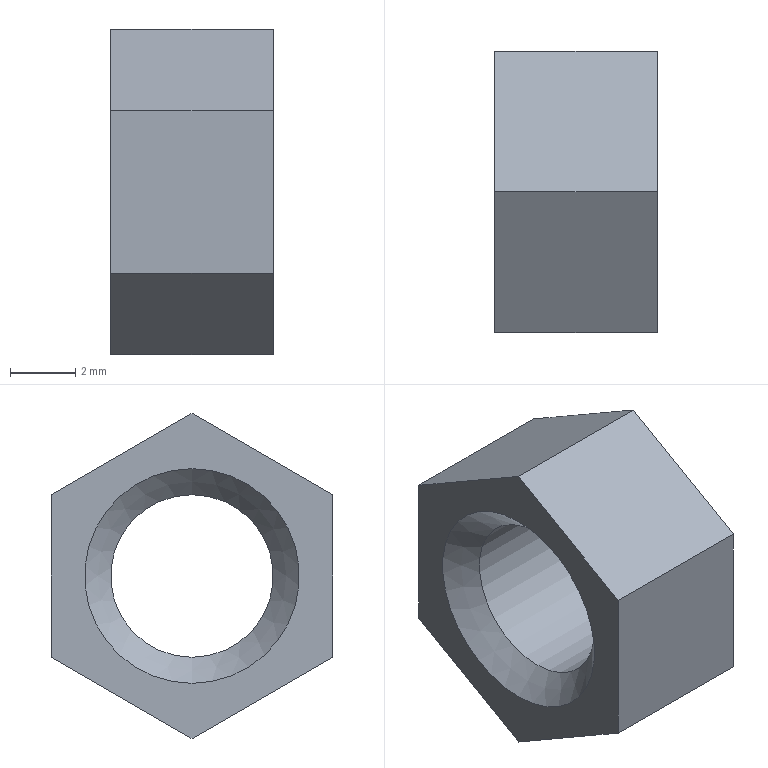Component | NX | ASSY_PRAC_PART_4 | 1 solid | 11 faces | box 5 x 8.66 x 10 mm | volume 215 mm3 | plane 8 | cone 2 | cylinder 1 | commonest cylinder face diameters 5 x1
STEP:
#1=CARTESIAN_POINT('',(0.,0.,0.));
#2=DIRECTION('',(0.,0.,1.));
#3=DIRECTION('',(1.,0.,0.));
#4=AXIS2_PLACEMENT_3D('',#1,#2,#3);
#5=CARTESIAN_POINT('',(18.5,0.3851,25.561));
#6=VERTEX_POINT('',#5);
#7=CARTESIAN_POINT('',(18.5,-3.945,23.061));
#8=VERTEX_POINT('',#7);
#9=CARTESIAN_POINT('',(18.5,0.3851,25.561));
#10=DIRECTION('',(0.,-0.866,-0.5));
#11=VECTOR('',#10,1.);
#12=LINE('',#9,#11);
#13=CARTESIAN_POINT('',(23.5,0.3851,25.561));
#14=DIRECTION('',(0.,0.5,-0.866));
#15=DIRECTION('',(0.,0.866,0.5));
#16=AXIS2_PLACEMENT_3D('',#13,#14,#15);
#17=PLANE('',#16);
#18=CARTESIAN_POINT('',(0.,-5.));
#19=DIRECTION('',(-1.,0.));
#20=VECTOR('',#19,1.);
#21=LINE('',#18,#20);
#22=(GEOMETRIC_REPRESENTATION_CONTEXT(2)PARAMETRIC_REPRESENTATION_CONTEXT()REPRESENTATION_CONTEXT('',''));
#23=DEFINITIONAL_REPRESENTATION('',(#21),#22);
#24=PCURVE('',#17,#23);
#25=CARTESIAN_POINT('',(18.5,0.3851,20.561));
#26=DIRECTION('',(1.,0.,0.));
#27=DIRECTION('',(0.,0.,-1.));
#28=AXIS2_PLACEMENT_3D('',#25,#26,#27);
#29=PLANE('',#28);
#30=CARTESIAN_POINT('',(-5.,0.));
#31=DIRECTION('',(0.5,-0.866));
#32=VECTOR('',#31,1.);
#33=LINE('',#30,#32);
#34=(GEOMETRIC_REPRESENTATION_CONTEXT(2)PARAMETRIC_REPRESENTATION_CONTEXT()REPRESENTATION_CONTEXT('',''));
#35=DEFINITIONAL_REPRESENTATION('',(#33),#34);
#36=PCURVE('',#29,#35);
#37=SURFACE_CURVE('',#12,(#24,#36),.PCURVE_S1.);
#38=EDGE_CURVE('',#6,#8,#37,.T.);
#39=ORIENTED_EDGE('',*,*,#38,.T.);
#40=CARTESIAN_POINT('',(23.5,-3.945,23.061));
#41=VERTEX_POINT('',#40);
#42=CARTESIAN_POINT('',(23.5,-3.945,23.061));
#43=DIRECTION('',(-1.,0.,0.));
#44=VECTOR('',#43,1.);
#45=LINE('',#42,#44);
#46=CARTESIAN_POINT('',(-5.,0.));
#47=DIRECTION('',(0.,-1.));
#48=VECTOR('',#47,1.);
#49=LINE('',#46,#48);
#50=(GEOMETRIC_REPRESENTATION_CONTEXT(2)PARAMETRIC_REPRESENTATION_CONTEXT()REPRESENTATION_CONTEXT('',''));
#51=DEFINITIONAL_REPRESENTATION('',(#49),#50);
#52=PCURVE('',#17,#51);
#53=CARTESIAN_POINT('',(23.5,-3.945,23.061));
#54=DIRECTION('',(0.,1.,-0.));
#55=DIRECTION('',(0.,0.,1.));
#56=AXIS2_PLACEMENT_3D('',#53,#54,#55);
#57=PLANE('',#56);
#58=CARTESIAN_POINT('',(0.,0.));
#59=DIRECTION('',(0.,-1.));
#60=VECTOR('',#59,1.);
#61=LINE('',#58,#60);
#62=(GEOMETRIC_REPRESENTATION_CONTEXT(2)PARAMETRIC_REPRESENTATION_CONTEXT()REPRESENTATION_CONTEXT('',''));
#63=DEFINITIONAL_REPRESENTATION('',(#61),#62);
#64=PCURVE('',#57,#63);
#65=SURFACE_CURVE('',#45,(#52,#64),.PCURVE_S1.);
#66=EDGE_CURVE('',#41,#8,#65,.T.);
#67=ORIENTED_EDGE('',*,*,#66,.F.);
#68=CARTESIAN_POINT('',(23.5,0.3851,25.561));
#69=VERTEX_POINT('',#68);
#70=CARTESIAN_POINT('',(23.5,0.3851,25.561));
#71=DIRECTION('',(0.,-0.866,-0.5));
#72=VECTOR('',#71,1.);
#73=LINE('',#70,#72);
#74=CARTESIAN_POINT('',(0.,0.));
#75=DIRECTION('',(-1.,0.));
#76=VECTOR('',#75,1.);
#77=LINE('',#74,#76);
#78=(GEOMETRIC_REPRESENTATION_CONTEXT(2)PARAMETRIC_REPRESENTATION_CONTEXT()REPRESENTATION_CONTEXT('',''));
#79=DEFINITIONAL_REPRESENTATION('',(#77),#78);
#80=PCURVE('',#17,#79);
#81=CARTESIAN_POINT('',(23.5,0.3851,20.561));
#82=DIRECTION('',(1.,0.,0.));
#83=DIRECTION('',(0.,0.,-1.));
#84=AXIS2_PLACEMENT_3D('',#81,#82,#83);
#85=PLANE('',#84);
#86=CARTESIAN_POINT('',(-5.,0.));
#87=DIRECTION('',(0.5,-0.866));
#88=VECTOR('',#87,1.);
#89=LINE('',#86,#88);
#90=(GEOMETRIC_REPRESENTATION_CONTEXT(2)PARAMETRIC_REPRESENTATION_CONTEXT()REPRESENTATION_CONTEXT('',''));
#91=DEFINITIONAL_REPRESENTATION('',(#89),#90);
#92=PCURVE('',#85,#91);
#93=SURFACE_CURVE('',#73,(#80,#92),.PCURVE_S1.);
#94=EDGE_CURVE('',#69,#41,#93,.T.);
#95=ORIENTED_EDGE('',*,*,#94,.F.);
#96=CARTESIAN_POINT('',(23.5,0.3851,25.561));
#97=DIRECTION('',(-1.,0.,0.));
#98=VECTOR('',#97,1.);
#99=LINE('',#96,#98);
#100=CARTESIAN_POINT('',(0.,0.));
#101=DIRECTION('',(0.,-1.));
#102=VECTOR('',#101,1.);
#103=LINE('',#100,#102);
#104=(GEOMETRIC_REPRESENTATION_CONTEXT(2)PARAMETRIC_REPRESENTATION_CONTEXT()REPRESENTATION_CONTEXT('',''));
#105=DEFINITIONAL_REPRESENTATION('',(#103),#104);
#106=PCURVE('',#17,#105);
#107=CARTESIAN_POINT('',(23.5,4.715,23.061));
#108=DIRECTION('',(0.,-0.5,-0.866));
#109=DIRECTION('',(0.,0.866,-0.5));
#110=AXIS2_PLACEMENT_3D('',#107,#108,#109);
#111=PLANE('',#110);
#112=CARTESIAN_POINT('',(-5.,0.));
#113=DIRECTION('',(0.,-1.));
#114=VECTOR('',#113,1.);
#115=LINE('',#112,#114);
#116=(GEOMETRIC_REPRESENTATION_CONTEXT(2)PARAMETRIC_REPRESENTATION_CONTEXT()REPRESENTATION_CONTEXT('',''));
#117=DEFINITIONAL_REPRESENTATION('',(#115),#116);
#118=PCURVE('',#111,#117);
#119=SURFACE_CURVE('',#99,(#106,#118),.PCURVE_S1.);
#120=EDGE_CURVE('',#69,#6,#119,.T.);
#121=ORIENTED_EDGE('',*,*,#120,.T.);
#122=EDGE_LOOP('',(#39,#67,#95,#121));
#123=FACE_BOUND('',#122,.T.);
#124=ADVANCED_FACE('',(#123),#17,.F.);
#125=CARTESIAN_POINT('',(18.5,-3.945,18.061));
#126=VERTEX_POINT('',#125);
#127=CARTESIAN_POINT('',(18.5,-3.945,23.061));
#128=DIRECTION('',(0.,-0.,-1.));
#129=VECTOR('',#128,1.);
#130=LINE('',#127,#129);
#131=CARTESIAN_POINT('',(0.,-5.));
#132=DIRECTION('',(-1.,0.));
#133=VECTOR('',#132,1.);
#134=LINE('',#131,#133);
#135=(GEOMETRIC_REPRESENTATION_CONTEXT(2)PARAMETRIC_REPRESENTATION_CONTEXT()REPRESENTATION_CONTEXT('',''));
#136=DEFINITIONAL_REPRESENTATION('',(#134),#135);
#137=PCURVE('',#57,#136);
#138=CARTESIAN_POINT('',(-2.5,-4.33));
#139=DIRECTION('',(1.,-0.));
#140=VECTOR('',#139,1.);
#141=LINE('',#138,#140);
#142=(GEOMETRIC_REPRESENTATION_CONTEXT(2)PARAMETRIC_REPRESENTATION_CONTEXT()REPRESENTATION_CONTEXT('',''));
#143=DEFINITIONAL_REPRESENTATION('',(#141),#142);
#144=PCURVE('',#29,#143);
#145=SURFACE_CURVE('',#130,(#137,#144),.PCURVE_S1.);
#146=EDGE_CURVE('',#8,#126,#145,.T.);
#147=ORIENTED_EDGE('',*,*,#146,.T.);
#148=CARTESIAN_POINT('',(23.5,-3.945,18.061));
#149=VERTEX_POINT('',#148);
#150=CARTESIAN_POINT('',(23.5,-3.945,18.061));
#151=DIRECTION('',(-1.,0.,0.));
#152=VECTOR('',#151,1.);
#153=LINE('',#150,#152);
#154=CARTESIAN_POINT('',(-5.,0.));
#155=DIRECTION('',(0.,-1.));
#156=VECTOR('',#155,1.);
#157=LINE('',#154,#156);
#158=(GEOMETRIC_REPRESENTATION_CONTEXT(2)PARAMETRIC_REPRESENTATION_CONTEXT()REPRESENTATION_CONTEXT('',''));
#159=DEFINITIONAL_REPRESENTATION('',(#157),#158);
#160=PCURVE('',#57,#159);
#161=CARTESIAN_POINT('',(23.5,-3.945,18.061));
#162=DIRECTION('',(0.,0.5,0.866));
#163=DIRECTION('',(0.,-0.866,0.5));
#164=AXIS2_PLACEMENT_3D('',#161,#162,#163);
#165=PLANE('',#164);
#166=CARTESIAN_POINT('',(0.,0.));
#167=DIRECTION('',(0.,-1.));
#168=VECTOR('',#167,1.);
#169=LINE('',#166,#168);
#170=(GEOMETRIC_REPRESENTATION_CONTEXT(2)PARAMETRIC_REPRESENTATION_CONTEXT()REPRESENTATION_CONTEXT('',''));
#171=DEFINITIONAL_REPRESENTATION('',(#169),#170);
#172=PCURVE('',#165,#171);
#173=SURFACE_CURVE('',#153,(#160,#172),.PCURVE_S1.);
#174=EDGE_CURVE('',#149,#126,#173,.T.);
#175=ORIENTED_EDGE('',*,*,#174,.F.);
#176=CARTESIAN_POINT('',(23.5,-3.945,23.061));
#177=DIRECTION('',(0.,-0.,-1.));
#178=VECTOR('',#177,1.);
#179=LINE('',#176,#178);
#180=CARTESIAN_POINT('',(0.,0.));
#181=DIRECTION('',(-1.,0.));
#182=VECTOR('',#181,1.);
#183=LINE('',#180,#182);
#184=(GEOMETRIC_REPRESENTATION_CONTEXT(2)PARAMETRIC_REPRESENTATION_CONTEXT()REPRESENTATION_CONTEXT('',''));
#185=DEFINITIONAL_REPRESENTATION('',(#183),#184);
#186=PCURVE('',#57,#185);
#187=CARTESIAN_POINT('',(-2.5,-4.33));
#188=DIRECTION('',(1.,-0.));
#189=VECTOR('',#188,1.);
#190=LINE('',#187,#189);
#191=(GEOMETRIC_REPRESENTATION_CONTEXT(2)PARAMETRIC_REPRESENTATION_CONTEXT()REPRESENTATION_CONTEXT('',''));
#192=DEFINITIONAL_REPRESENTATION('',(#190),#191);
#193=PCURVE('',#85,#192);
#194=SURFACE_CURVE('',#179,(#186,#193),.PCURVE_S1.);
#195=EDGE_CURVE('',#41,#149,#194,.T.);
#196=ORIENTED_EDGE('',*,*,#195,.F.);
#197=ORIENTED_EDGE('',*,*,#66,.T.);
#198=EDGE_LOOP('',(#147,#175,#196,#197));
#199=FACE_BOUND('',#198,.T.);
#200=ADVANCED_FACE('',(#199),#57,.F.);
#201=CARTESIAN_POINT('',(18.5,0.3851,15.561));
#202=VERTEX_POINT('',#201);
#203=CARTESIAN_POINT('',(18.5,-3.945,18.061));
#204=DIRECTION('',(0.,0.866,-0.5));
#205=VECTOR('',#204,1.);
#206=LINE('',#203,#205);
#207=CARTESIAN_POINT('',(0.,-5.));
#208=DIRECTION('',(-1.,0.));
#209=VECTOR('',#208,1.);
#210=LINE('',#207,#209);
#211=(GEOMETRIC_REPRESENTATION_CONTEXT(2)PARAMETRIC_REPRESENTATION_CONTEXT()REPRESENTATION_CONTEXT('',''));
#212=DEFINITIONAL_REPRESENTATION('',(#210),#211);
#213=PCURVE('',#165,#212);
#214=CARTESIAN_POINT('',(2.5,-4.33));
#215=DIRECTION('',(0.5,0.866));
#216=VECTOR('',#215,1.);
#217=LINE('',#214,#216);
#218=(GEOMETRIC_REPRESENTATION_CONTEXT(2)PARAMETRIC_REPRESENTATION_CONTEXT()REPRESENTATION_CONTEXT('',''));
#219=DEFINITIONAL_REPRESENTATION('',(#217),#218);
#220=PCURVE('',#29,#219);
#221=SURFACE_CURVE('',#206,(#213,#220),.PCURVE_S1.);
#222=EDGE_CURVE('',#126,#202,#221,.T.);
#223=ORIENTED_EDGE('',*,*,#222,.T.);
#224=CARTESIAN_POINT('',(23.5,0.3851,15.561));
#225=VERTEX_POINT('',#224);
#226=CARTESIAN_POINT('',(23.5,0.3851,15.561));
#227=DIRECTION('',(-1.,0.,0.));
#228=VECTOR('',#227,1.);
#229=LINE('',#226,#228);
#230=CARTESIAN_POINT('',(-5.,0.));
#231=DIRECTION('',(0.,-1.));
#232=VECTOR('',#231,1.);
#233=LINE('',#230,#232);
#234=(GEOMETRIC_REPRESENTATION_CONTEXT(2)PARAMETRIC_REPRESENTATION_CONTEXT()REPRESENTATION_CONTEXT('',''));
#235=DEFINITIONAL_REPRESENTATION('',(#233),#234);
#236=PCURVE('',#165,#235);
#237=CARTESIAN_POINT('',(23.5,0.3851,15.561));
#238=DIRECTION('',(0.,-0.5,0.866));
#239=DIRECTION('',(0.,-0.866,-0.5));
#240=AXIS2_PLACEMENT_3D('',#237,#238,#239);
#241=PLANE('',#240);
#242=CARTESIAN_POINT('',(0.,0.));
#243=DIRECTION('',(0.,-1.));
#244=VECTOR('',#243,1.);
#245=LINE('',#242,#244);
#246=(GEOMETRIC_REPRESENTATION_CONTEXT(2)PARAMETRIC_REPRESENTATION_CONTEXT()REPRESENTATION_CONTEXT('',''));
#247=DEFINITIONAL_REPRESENTATION('',(#245),#246);
#248=PCURVE('',#241,#247);
#249=SURFACE_CURVE('',#229,(#236,#248),.PCURVE_S1.);
#250=EDGE_CURVE('',#225,#202,#249,.T.);
#251=ORIENTED_EDGE('',*,*,#250,.F.);
#252=CARTESIAN_POINT('',(23.5,-3.945,18.061));
#253=DIRECTION('',(0.,0.866,-0.5));
#254=VECTOR('',#253,1.);
#255=LINE('',#252,#254);
#256=CARTESIAN_POINT('',(0.,0.));
#257=DIRECTION('',(-1.,0.));
#258=VECTOR('',#257,1.);
#259=LINE('',#256,#258);
#260=(GEOMETRIC_REPRESENTATION_CONTEXT(2)PARAMETRIC_REPRESENTATION_CONTEXT()REPRESENTATION_CONTEXT('',''));
#261=DEFINITIONAL_REPRESENTATION('',(#259),#260);
#262=PCURVE('',#165,#261);
#263=CARTESIAN_POINT('',(2.5,-4.33));
#264=DIRECTION('',(0.5,0.866));
#265=VECTOR('',#264,1.);
#266=LINE('',#263,#265);
#267=(GEOMETRIC_REPRESENTATION_CONTEXT(2)PARAMETRIC_REPRESENTATION_CONTEXT()REPRESENTATION_CONTEXT('',''));
#268=DEFINITIONAL_REPRESENTATION('',(#266),#267);
#269=PCURVE('',#85,#268);
#270=SURFACE_CURVE('',#255,(#262,#269),.PCURVE_S1.);
#271=EDGE_CURVE('',#149,#225,#270,.T.);
#272=ORIENTED_EDGE('',*,*,#271,.F.);
#273=ORIENTED_EDGE('',*,*,#174,.T.);
#274=EDGE_LOOP('',(#223,#251,#272,#273));
#275=FACE_BOUND('',#274,.T.);
#276=ADVANCED_FACE('',(#275),#165,.F.);
#277=CARTESIAN_POINT('',(18.5,4.715,18.061));
#278=VERTEX_POINT('',#277);
#279=CARTESIAN_POINT('',(18.5,0.3851,15.561));
#280=DIRECTION('',(0.,0.866,0.5));
#281=VECTOR('',#280,1.);
#282=LINE('',#279,#281);
#283=CARTESIAN_POINT('',(0.,-5.));
#284=DIRECTION('',(-1.,0.));
#285=VECTOR('',#284,1.);
#286=LINE('',#283,#285);
#287=(GEOMETRIC_REPRESENTATION_CONTEXT(2)PARAMETRIC_REPRESENTATION_CONTEXT()REPRESENTATION_CONTEXT('',''));
#288=DEFINITIONAL_REPRESENTATION('',(#286),#287);
#289=PCURVE('',#241,#288);
#290=CARTESIAN_POINT('',(5.,-0.));
#291=DIRECTION('',(-0.5,0.866));
#292=VECTOR('',#291,1.);
#293=LINE('',#290,#292);
#294=(GEOMETRIC_REPRESENTATION_CONTEXT(2)PARAMETRIC_REPRESENTATION_CONTEXT()REPRESENTATION_CONTEXT('',''));
#295=DEFINITIONAL_REPRESENTATION('',(#293),#294);
#296=PCURVE('',#29,#295);
#297=SURFACE_CURVE('',#282,(#289,#296),.PCURVE_S1.);
#298=EDGE_CURVE('',#202,#278,#297,.T.);
#299=ORIENTED_EDGE('',*,*,#298,.T.);
#300=CARTESIAN_POINT('',(23.5,4.715,18.061));
#301=VERTEX_POINT('',#300);
#302=CARTESIAN_POINT('',(23.5,4.715,18.061));
#303=DIRECTION('',(-1.,0.,0.));
#304=VECTOR('',#303,1.);
#305=LINE('',#302,#304);
#306=CARTESIAN_POINT('',(-5.,0.));
#307=DIRECTION('',(0.,-1.));
#308=VECTOR('',#307,1.);
#309=LINE('',#306,#308);
#310=(GEOMETRIC_REPRESENTATION_CONTEXT(2)PARAMETRIC_REPRESENTATION_CONTEXT()REPRESENTATION_CONTEXT('',''));
#311=DEFINITIONAL_REPRESENTATION('',(#309),#310);
#312=PCURVE('',#241,#311);
#313=CARTESIAN_POINT('',(23.5,4.715,18.061));
#314=DIRECTION('',(0.,-1.,0.));
#315=DIRECTION('',(0.,-0.,-1.));
#316=AXIS2_PLACEMENT_3D('',#313,#314,#315);
#317=PLANE('',#316);
#318=CARTESIAN_POINT('',(0.,0.));
#319=DIRECTION('',(0.,-1.));
#320=VECTOR('',#319,1.);
#321=LINE('',#318,#320);
#322=(GEOMETRIC_REPRESENTATION_CONTEXT(2)PARAMETRIC_REPRESENTATION_CONTEXT()REPRESENTATION_CONTEXT('',''));
#323=DEFINITIONAL_REPRESENTATION('',(#321),#322);
#324=PCURVE('',#317,#323);
#325=SURFACE_CURVE('',#305,(#312,#324),.PCURVE_S1.);
#326=EDGE_CURVE('',#301,#278,#325,.T.);
#327=ORIENTED_EDGE('',*,*,#326,.F.);
#328=CARTESIAN_POINT('',(23.5,0.3851,15.561));
#329=DIRECTION('',(0.,0.866,0.5));
#330=VECTOR('',#329,1.);
#331=LINE('',#328,#330);
#332=CARTESIAN_POINT('',(0.,0.));
#333=DIRECTION('',(-1.,0.));
#334=VECTOR('',#333,1.);
#335=LINE('',#332,#334);
#336=(GEOMETRIC_REPRESENTATION_CONTEXT(2)PARAMETRIC_REPRESENTATION_CONTEXT()REPRESENTATION_CONTEXT('',''));
#337=DEFINITIONAL_REPRESENTATION('',(#335),#336);
#338=PCURVE('',#241,#337);
#339=CARTESIAN_POINT('',(5.,-0.));
#340=DIRECTION('',(-0.5,0.866));
#341=VECTOR('',#340,1.);
#342=LINE('',#339,#341);
#343=(GEOMETRIC_REPRESENTATION_CONTEXT(2)PARAMETRIC_REPRESENTATION_CONTEXT()REPRESENTATION_CONTEXT('',''));
#344=DEFINITIONAL_REPRESENTATION('',(#342),#343);
#345=PCURVE('',#85,#344);
#346=SURFACE_CURVE('',#331,(#338,#345),.PCURVE_S1.);
#347=EDGE_CURVE('',#225,#301,#346,.T.);
#348=ORIENTED_EDGE('',*,*,#347,.F.);
#349=ORIENTED_EDGE('',*,*,#250,.T.);
#350=EDGE_LOOP('',(#299,#327,#348,#349));
#351=FACE_BOUND('',#350,.T.);
#352=ADVANCED_FACE('',(#351),#241,.F.);
#353=CARTESIAN_POINT('',(18.5,4.715,23.061));
#354=VERTEX_POINT('',#353);
#355=CARTESIAN_POINT('',(18.5,4.715,18.061));
#356=DIRECTION('',(0.,0.,1.));
#357=VECTOR('',#356,1.);
#358=LINE('',#355,#357);
#359=CARTESIAN_POINT('',(0.,-5.));
#360=DIRECTION('',(-1.,0.));
#361=VECTOR('',#360,1.);
#362=LINE('',#359,#361);
#363=(GEOMETRIC_REPRESENTATION_CONTEXT(2)PARAMETRIC_REPRESENTATION_CONTEXT()REPRESENTATION_CONTEXT('',''));
#364=DEFINITIONAL_REPRESENTATION('',(#362),#363);
#365=PCURVE('',#317,#364);
#366=CARTESIAN_POINT('',(2.5,4.33));
#367=DIRECTION('',(-1.,0.));
#368=VECTOR('',#367,1.);
#369=LINE('',#366,#368);
#370=(GEOMETRIC_REPRESENTATION_CONTEXT(2)PARAMETRIC_REPRESENTATION_CONTEXT()REPRESENTATION_CONTEXT('',''));
#371=DEFINITIONAL_REPRESENTATION('',(#369),#370);
#372=PCURVE('',#29,#371);
#373=SURFACE_CURVE('',#358,(#365,#372),.PCURVE_S1.);
#374=EDGE_CURVE('',#278,#354,#373,.T.);
#375=ORIENTED_EDGE('',*,*,#374,.T.);
#376=CARTESIAN_POINT('',(23.5,4.715,23.061));
#377=VERTEX_POINT('',#376);
#378=CARTESIAN_POINT('',(23.5,4.715,23.061));
#379=DIRECTION('',(-1.,0.,0.));
#380=VECTOR('',#379,1.);
#381=LINE('',#378,#380);
#382=CARTESIAN_POINT('',(-5.,0.));
#383=DIRECTION('',(0.,-1.));
#384=VECTOR('',#383,1.);
#385=LINE('',#382,#384);
#386=(GEOMETRIC_REPRESENTATION_CONTEXT(2)PARAMETRIC_REPRESENTATION_CONTEXT()REPRESENTATION_CONTEXT('',''));
#387=DEFINITIONAL_REPRESENTATION('',(#385),#386);
#388=PCURVE('',#317,#387);
#389=CARTESIAN_POINT('',(0.,0.));
#390=DIRECTION('',(0.,-1.));
#391=VECTOR('',#390,1.);
#392=LINE('',#389,#391);
#393=(GEOMETRIC_REPRESENTATION_CONTEXT(2)PARAMETRIC_REPRESENTATION_CONTEXT()REPRESENTATION_CONTEXT('',''));
#394=DEFINITIONAL_REPRESENTATION('',(#392),#393);
#395=PCURVE('',#111,#394);
#396=SURFACE_CURVE('',#381,(#388,#395),.PCURVE_S1.);
#397=EDGE_CURVE('',#377,#354,#396,.T.);
#398=ORIENTED_EDGE('',*,*,#397,.F.);
#399=CARTESIAN_POINT('',(23.5,4.715,18.061));
#400=DIRECTION('',(0.,0.,1.));
#401=VECTOR('',#400,1.);
#402=LINE('',#399,#401);
#403=CARTESIAN_POINT('',(0.,0.));
#404=DIRECTION('',(-1.,0.));
#405=VECTOR('',#404,1.);
#406=LINE('',#403,#405);
#407=(GEOMETRIC_REPRESENTATION_CONTEXT(2)PARAMETRIC_REPRESENTATION_CONTEXT()REPRESENTATION_CONTEXT('',''));
#408=DEFINITIONAL_REPRESENTATION('',(#406),#407);
#409=PCURVE('',#317,#408);
#410=CARTESIAN_POINT('',(2.5,4.33));
#411=DIRECTION('',(-1.,0.));
#412=VECTOR('',#411,1.);
#413=LINE('',#410,#412);
#414=(GEOMETRIC_REPRESENTATION_CONTEXT(2)PARAMETRIC_REPRESENTATION_CONTEXT()REPRESENTATION_CONTEXT('',''));
#415=DEFINITIONAL_REPRESENTATION('',(#413),#414);
#416=PCURVE('',#85,#415);
#417=SURFACE_CURVE('',#402,(#409,#416),.PCURVE_S1.);
#418=EDGE_CURVE('',#301,#377,#417,.T.);
#419=ORIENTED_EDGE('',*,*,#418,.F.);
#420=ORIENTED_EDGE('',*,*,#326,.T.);
#421=EDGE_LOOP('',(#375,#398,#419,#420));
#422=FACE_BOUND('',#421,.T.);
#423=ADVANCED_FACE('',(#422),#317,.F.);
#424=CARTESIAN_POINT('',(18.5,4.715,23.061));
#425=DIRECTION('',(0.,-0.866,0.5));
#426=VECTOR('',#425,1.);
#427=LINE('',#424,#426);
#428=CARTESIAN_POINT('',(0.,-5.));
#429=DIRECTION('',(-1.,0.));
#430=VECTOR('',#429,1.);
#431=LINE('',#428,#430);
#432=(GEOMETRIC_REPRESENTATION_CONTEXT(2)PARAMETRIC_REPRESENTATION_CONTEXT()REPRESENTATION_CONTEXT('',''));
#433=DEFINITIONAL_REPRESENTATION('',(#431),#432);
#434=PCURVE('',#111,#433);
#435=CARTESIAN_POINT('',(-2.5,4.33));
#436=DIRECTION('',(-0.5,-0.866));
#437=VECTOR('',#436,1.);
#438=LINE('',#435,#437);
#439=(GEOMETRIC_REPRESENTATION_CONTEXT(2)PARAMETRIC_REPRESENTATION_CONTEXT()REPRESENTATION_CONTEXT('',''));
#440=DEFINITIONAL_REPRESENTATION('',(#438),#439);
#441=PCURVE('',#29,#440);
#442=SURFACE_CURVE('',#427,(#434,#441),.PCURVE_S1.);
#443=EDGE_CURVE('',#354,#6,#442,.T.);
#444=ORIENTED_EDGE('',*,*,#443,.T.);
#445=ORIENTED_EDGE('',*,*,#120,.F.);
#446=CARTESIAN_POINT('',(23.5,4.715,23.061));
#447=DIRECTION('',(0.,-0.866,0.5));
#448=VECTOR('',#447,1.);
#449=LINE('',#446,#448);
#450=CARTESIAN_POINT('',(0.,0.));
#451=DIRECTION('',(-1.,0.));
#452=VECTOR('',#451,1.);
#453=LINE('',#450,#452);
#454=(GEOMETRIC_REPRESENTATION_CONTEXT(2)PARAMETRIC_REPRESENTATION_CONTEXT()REPRESENTATION_CONTEXT('',''));
#455=DEFINITIONAL_REPRESENTATION('',(#453),#454);
#456=PCURVE('',#111,#455);
#457=CARTESIAN_POINT('',(-2.5,4.33));
#458=DIRECTION('',(-0.5,-0.866));
#459=VECTOR('',#458,1.);
#460=LINE('',#457,#459);
#461=(GEOMETRIC_REPRESENTATION_CONTEXT(2)PARAMETRIC_REPRESENTATION_CONTEXT()REPRESENTATION_CONTEXT('',''));
#462=DEFINITIONAL_REPRESENTATION('',(#460),#461);
#463=PCURVE('',#85,#462);
#464=SURFACE_CURVE('',#449,(#456,#463),.PCURVE_S1.);
#465=EDGE_CURVE('',#377,#69,#464,.T.);
#466=ORIENTED_EDGE('',*,*,#465,.F.);
#467=ORIENTED_EDGE('',*,*,#397,.T.);
#468=EDGE_LOOP('',(#444,#445,#466,#467));
#469=FACE_BOUND('',#468,.T.);
#470=ADVANCED_FACE('',(#469),#111,.F.);
#471=CARTESIAN_POINT('',(23.5,0.3851,17.261));
#472=VERTEX_POINT('',#471);
#473=CARTESIAN_POINT('',(23.5,0.3851,20.561));
#474=DIRECTION('',(-1.,0.,0.));
#475=DIRECTION('',(0.,0.,-1.));
#476=AXIS2_PLACEMENT_3D('',#473,#474,#475);
#477=CIRCLE('',#476,3.3);
#478=CARTESIAN_POINT('',(3.3,0.));
#479=CARTESIAN_POINT('',(3.3,-5.716));
#480=CARTESIAN_POINT('',(-1.65,-2.858));
#481=CARTESIAN_POINT('',(-6.6,-0.));
#482=CARTESIAN_POINT('',(-1.65,2.858));
#483=CARTESIAN_POINT('',(3.3,5.716));
#484=CARTESIAN_POINT('',(3.3,0.));
#485=(BOUNDED_CURVE()B_SPLINE_CURVE(2,(#478,#479,#480,#481,#482,#483,#484),.UNSPECIFIED.,.T.,.F.)B_SPLINE_CURVE_WITH_KNOTS((1,2,2,2,2,1),(-2.094,0.,2.094,4.189,6.283,8.378),.UNSPECIFIED.)CURVE()GEOMETRIC_REPRESENTATION_ITEM()RATIONAL_B_SPLINE_CURVE((1.,0.5,1.,0.5,1.,0.5,1.))REPRESENTATION_ITEM(''));
#486=(GEOMETRIC_REPRESENTATION_CONTEXT(2)PARAMETRIC_REPRESENTATION_CONTEXT()REPRESENTATION_CONTEXT('',''));
#487=DEFINITIONAL_REPRESENTATION('',(#485),#486);
#488=PCURVE('',#85,#487);
#489=CARTESIAN_POINT('',(22.7,0.3851,20.561));
#490=DIRECTION('',(1.,0.,0.));
#491=DIRECTION('',(0.,0.,-1.));
#492=AXIS2_PLACEMENT_3D('',#489,#490,#491);
#493=CONICAL_SURFACE('',#492,2.5,0.7854);
#494=CARTESIAN_POINT('',(6.283,0.8));
#495=DIRECTION('',(-1.,0.));
#496=VECTOR('',#495,1.);
#497=LINE('',#494,#496);
#498=(GEOMETRIC_REPRESENTATION_CONTEXT(2)PARAMETRIC_REPRESENTATION_CONTEXT()REPRESENTATION_CONTEXT('',''));
#499=DEFINITIONAL_REPRESENTATION('',(#497),#498);
#500=PCURVE('',#493,#499);
#501=SURFACE_CURVE('',#477,(#488,#500),.PCURVE_S1.);
#502=EDGE_CURVE('',#472,#472,#501,.T.);
#503=ORIENTED_EDGE('',*,*,#502,.T.);
#504=EDGE_LOOP('',(#503));
#505=FACE_BOUND('',#504,.T.);
#506=ORIENTED_EDGE('',*,*,#94,.T.);
#507=ORIENTED_EDGE('',*,*,#195,.T.);
#508=ORIENTED_EDGE('',*,*,#271,.T.);
#509=ORIENTED_EDGE('',*,*,#347,.T.);
#510=ORIENTED_EDGE('',*,*,#418,.T.);
#511=ORIENTED_EDGE('',*,*,#465,.T.);
#512=EDGE_LOOP('',(#506,#507,#508,#509,#510,#511));
#513=FACE_BOUND('',#512,.T.);
#514=ADVANCED_FACE('',(#505,#513),#85,.T.);
#515=CARTESIAN_POINT('',(18.5,0.3851,17.261));
#516=VERTEX_POINT('',#515);
#517=CARTESIAN_POINT('',(18.5,0.3851,20.561));
#518=DIRECTION('',(1.,0.,0.));
#519=DIRECTION('',(0.,0.,-1.));
#520=AXIS2_PLACEMENT_3D('',#517,#518,#519);
#521=CIRCLE('',#520,3.3);
#522=CARTESIAN_POINT('',(0.,0.));
#523=DIRECTION('',(1.,0.));
#524=AXIS2_PLACEMENT_2D('',#522,#523);
#525=CIRCLE('',#524,3.3);
#526=(GEOMETRIC_REPRESENTATION_CONTEXT(2)PARAMETRIC_REPRESENTATION_CONTEXT()REPRESENTATION_CONTEXT('',''));
#527=DEFINITIONAL_REPRESENTATION('',(#525),#526);
#528=PCURVE('',#29,#527);
#529=CARTESIAN_POINT('',(18.5,0.3851,20.561));
#530=DIRECTION('',(-1.,0.,0.));
#531=DIRECTION('',(0.,0.,1.));
#532=AXIS2_PLACEMENT_3D('',#529,#530,#531);
#533=CONICAL_SURFACE('',#532,3.3,0.7854);
#534=CARTESIAN_POINT('',(9.425,0.));
#535=DIRECTION('',(-1.,0.));
#536=VECTOR('',#535,1.);
#537=LINE('',#534,#536);
#538=(GEOMETRIC_REPRESENTATION_CONTEXT(2)PARAMETRIC_REPRESENTATION_CONTEXT()REPRESENTATION_CONTEXT('',''));
#539=DEFINITIONAL_REPRESENTATION('',(#537),#538);
#540=PCURVE('',#533,#539);
#541=SURFACE_CURVE('',#521,(#528,#540),.PCURVE_S1.);
#542=EDGE_CURVE('',#516,#516,#541,.T.);
#543=ORIENTED_EDGE('',*,*,#542,.T.);
#544=EDGE_LOOP('',(#543));
#545=FACE_BOUND('',#544,.T.);
#546=ORIENTED_EDGE('',*,*,#38,.F.);
#547=ORIENTED_EDGE('',*,*,#443,.F.);
#548=ORIENTED_EDGE('',*,*,#374,.F.);
#549=ORIENTED_EDGE('',*,*,#298,.F.);
#550=ORIENTED_EDGE('',*,*,#222,.F.);
#551=ORIENTED_EDGE('',*,*,#146,.F.);
#552=EDGE_LOOP('',(#546,#547,#548,#549,#550,#551));
#553=FACE_BOUND('',#552,.T.);
#554=ADVANCED_FACE('',(#545,#553),#29,.F.);
#555=CARTESIAN_POINT('',(22.7,0.3851,18.061));
#556=VERTEX_POINT('',#555);
#557=CARTESIAN_POINT('',(22.7,0.3851,20.561));
#558=DIRECTION('',(1.,0.,0.));
#559=DIRECTION('',(0.,0.,-1.));
#560=AXIS2_PLACEMENT_3D('',#557,#558,#559);
#561=CIRCLE('',#560,2.5);
#562=CARTESIAN_POINT('',(18.5,0.3851,20.561));
#563=DIRECTION('',(1.,0.,0.));
#564=DIRECTION('',(0.,0.,-1.));
#565=AXIS2_PLACEMENT_3D('',#562,#563,#564);
#566=CYLINDRICAL_SURFACE('',#565,2.5);
#567=CARTESIAN_POINT('',(0.,4.2));
#568=DIRECTION('',(1.,0.));
#569=VECTOR('',#568,1.);
#570=LINE('',#567,#569);
#571=(GEOMETRIC_REPRESENTATION_CONTEXT(2)PARAMETRIC_REPRESENTATION_CONTEXT()REPRESENTATION_CONTEXT('',''));
#572=DEFINITIONAL_REPRESENTATION('',(#570),#571);
#573=PCURVE('',#566,#572);
#574=CARTESIAN_POINT('',(0.,0.));
#575=DIRECTION('',(1.,0.));
#576=VECTOR('',#575,1.);
#577=LINE('',#574,#576);
#578=(GEOMETRIC_REPRESENTATION_CONTEXT(2)PARAMETRIC_REPRESENTATION_CONTEXT()REPRESENTATION_CONTEXT('',''));
#579=DEFINITIONAL_REPRESENTATION('',(#577),#578);
#580=PCURVE('',#493,#579);
#581=SURFACE_CURVE('',#561,(#573,#580),.PCURVE_S1.);
#582=EDGE_CURVE('',#556,#556,#581,.T.);
#583=ORIENTED_EDGE('',*,*,#582,.F.);
#584=CARTESIAN_POINT('',(19.3,0.3851,18.061));
#585=VERTEX_POINT('',#584);
#586=CARTESIAN_POINT('',(19.3,0.3851,18.061));
#587=CARTESIAN_POINT('',(22.7,0.3851,18.061));
#588=B_SPLINE_CURVE_WITH_KNOTS('',1,(#586,#587),.UNSPECIFIED.,.F.,.F.,(2,2),(0.8,4.2),.PIECEWISE_BEZIER_KNOTS.);
#589=CARTESIAN_POINT('',(0.,0.));
#590=DIRECTION('',(0.,1.));
#591=VECTOR('',#590,1.);
#592=LINE('',#589,#591);
#593=(GEOMETRIC_REPRESENTATION_CONTEXT(2)PARAMETRIC_REPRESENTATION_CONTEXT()REPRESENTATION_CONTEXT('',''));
#594=DEFINITIONAL_REPRESENTATION('',(#592),#593);
#595=PCURVE('',#566,#594);
#596=CARTESIAN_POINT('',(6.283,0.));
#597=DIRECTION('',(0.,1.));
#598=VECTOR('',#597,1.);
#599=LINE('',#596,#598);
#600=(GEOMETRIC_REPRESENTATION_CONTEXT(2)PARAMETRIC_REPRESENTATION_CONTEXT()REPRESENTATION_CONTEXT('',''));
#601=DEFINITIONAL_REPRESENTATION('',(#599),#600);
#602=PCURVE('',#566,#601);
#603=SEAM_CURVE('',#588,(#595,#602),.PCURVE_S1.);
#604=EDGE_CURVE('',#585,#556,#603,.T.);
#605=ORIENTED_EDGE('',*,*,#604,.F.);
#606=CARTESIAN_POINT('',(19.3,0.3851,20.561));
#607=DIRECTION('',(-1.,0.,0.));
#608=DIRECTION('',(0.,0.,-1.));
#609=AXIS2_PLACEMENT_3D('',#606,#607,#608);
#610=CIRCLE('',#609,2.5);
#611=CARTESIAN_POINT('',(6.283,0.8));
#612=DIRECTION('',(-1.,0.));
#613=VECTOR('',#612,1.);
#614=LINE('',#611,#613);
#615=(GEOMETRIC_REPRESENTATION_CONTEXT(2)PARAMETRIC_REPRESENTATION_CONTEXT()REPRESENTATION_CONTEXT('',''));
#616=DEFINITIONAL_REPRESENTATION('',(#614),#615);
#617=PCURVE('',#566,#616);
#618=CARTESIAN_POINT('',(3.142,-0.8));
#619=DIRECTION('',(1.,0.));
#620=VECTOR('',#619,1.);
#621=LINE('',#618,#620);
#622=(GEOMETRIC_REPRESENTATION_CONTEXT(2)PARAMETRIC_REPRESENTATION_CONTEXT()REPRESENTATION_CONTEXT('',''));
#623=DEFINITIONAL_REPRESENTATION('',(#621),#622);
#624=PCURVE('',#533,#623);
#625=SURFACE_CURVE('',#610,(#617,#624),.PCURVE_S1.);
#626=EDGE_CURVE('',#585,#585,#625,.T.);
#627=ORIENTED_EDGE('',*,*,#626,.F.);
#628=ORIENTED_EDGE('',*,*,#604,.T.);
#629=EDGE_LOOP('',(#583,#605,#627,#628));
#630=FACE_BOUND('',#629,.F.);
#631=ADVANCED_FACE('',(#630),#566,.F.);
#632=ORIENTED_EDGE('',*,*,#626,.T.);
#633=CARTESIAN_POINT('',(19.3,0.3851,18.061));
#634=CARTESIAN_POINT('',(18.5,0.3851,17.261));
#635=B_SPLINE_CURVE_WITH_KNOTS('',1,(#633,#634),.UNSPECIFIED.,.F.,.F.,(2,2),(-1.131,0.),.PIECEWISE_BEZIER_KNOTS.);
#636=CARTESIAN_POINT('',(9.425,0.));
#637=DIRECTION('',(0.,1.));
#638=VECTOR('',#637,1.);
#639=LINE('',#636,#638);
#640=(GEOMETRIC_REPRESENTATION_CONTEXT(2)PARAMETRIC_REPRESENTATION_CONTEXT()REPRESENTATION_CONTEXT('',''));
#641=DEFINITIONAL_REPRESENTATION('',(#639),#640);
#642=PCURVE('',#533,#641);
#643=CARTESIAN_POINT('',(3.142,0.));
#644=DIRECTION('',(0.,1.));
#645=VECTOR('',#644,1.);
#646=LINE('',#643,#645);
#647=(GEOMETRIC_REPRESENTATION_CONTEXT(2)PARAMETRIC_REPRESENTATION_CONTEXT()REPRESENTATION_CONTEXT('',''));
#648=DEFINITIONAL_REPRESENTATION('',(#646),#647);
#649=PCURVE('',#533,#648);
#650=SEAM_CURVE('',#635,(#642,#649),.PCURVE_S1.);
#651=EDGE_CURVE('',#585,#516,#650,.T.);
#652=ORIENTED_EDGE('',*,*,#651,.T.);
#653=ORIENTED_EDGE('',*,*,#542,.T.);
#654=ORIENTED_EDGE('',*,*,#651,.F.);
#655=EDGE_LOOP('',(#632,#652,#653,#654));
#656=FACE_BOUND('',#655,.F.);
#657=ADVANCED_FACE('',(#656),#533,.F.);
#658=ORIENTED_EDGE('',*,*,#502,.T.);
#659=CARTESIAN_POINT('',(22.7,0.3851,18.061));
#660=CARTESIAN_POINT('',(23.5,0.3851,17.261));
#661=B_SPLINE_CURVE_WITH_KNOTS('',1,(#659,#660),.UNSPECIFIED.,.F.,.F.,(2,2),(0.,1.131),.PIECEWISE_BEZIER_KNOTS.);
#662=CARTESIAN_POINT('',(0.,0.));
#663=DIRECTION('',(0.,1.));
#664=VECTOR('',#663,1.);
#665=LINE('',#662,#664);
#666=(GEOMETRIC_REPRESENTATION_CONTEXT(2)PARAMETRIC_REPRESENTATION_CONTEXT()REPRESENTATION_CONTEXT('',''));
#667=DEFINITIONAL_REPRESENTATION('',(#665),#666);
#668=PCURVE('',#493,#667);
#669=CARTESIAN_POINT('',(6.283,0.));
#670=DIRECTION('',(0.,1.));
#671=VECTOR('',#670,1.);
#672=LINE('',#669,#671);
#673=(GEOMETRIC_REPRESENTATION_CONTEXT(2)PARAMETRIC_REPRESENTATION_CONTEXT()REPRESENTATION_CONTEXT('',''));
#674=DEFINITIONAL_REPRESENTATION('',(#672),#673);
#675=PCURVE('',#493,#674);
#676=SEAM_CURVE('',#661,(#668,#675),.PCURVE_S1.);
#677=EDGE_CURVE('',#556,#472,#676,.T.);
#678=ORIENTED_EDGE('',*,*,#677,.F.);
#679=ORIENTED_EDGE('',*,*,#582,.T.);
#680=ORIENTED_EDGE('',*,*,#677,.T.);
#681=EDGE_LOOP('',(#658,#678,#679,#680));
#682=FACE_BOUND('',#681,.F.);
#683=ADVANCED_FACE('',(#682),#493,.F.);
#684=CLOSED_SHELL('',(#124,#200,#276,#352,#423,#470,#514,#554,#631,#657,#683));
#685=MANIFOLD_SOLID_BREP('',#684);
#686=(LENGTH_UNIT()NAMED_UNIT(*)SI_UNIT(.MILLI.,.METRE.));
#687=UNCERTAINTY_MEASURE_WITH_UNIT(LENGTH_MEASURE(0.000002),#686,'','');
#688=(NAMED_UNIT(*)PLANE_ANGLE_UNIT()SI_UNIT($,.RADIAN.));
#689=(NAMED_UNIT(*)SI_UNIT($,.STERADIAN.)SOLID_ANGLE_UNIT());
#690=(GEOMETRIC_REPRESENTATION_CONTEXT(3)GLOBAL_UNCERTAINTY_ASSIGNED_CONTEXT((#687))GLOBAL_UNIT_ASSIGNED_CONTEXT((#686,#688,#689))REPRESENTATION_CONTEXT('',''));
#691=ADVANCED_BREP_SHAPE_REPRESENTATION('',(#4,#685),#690);